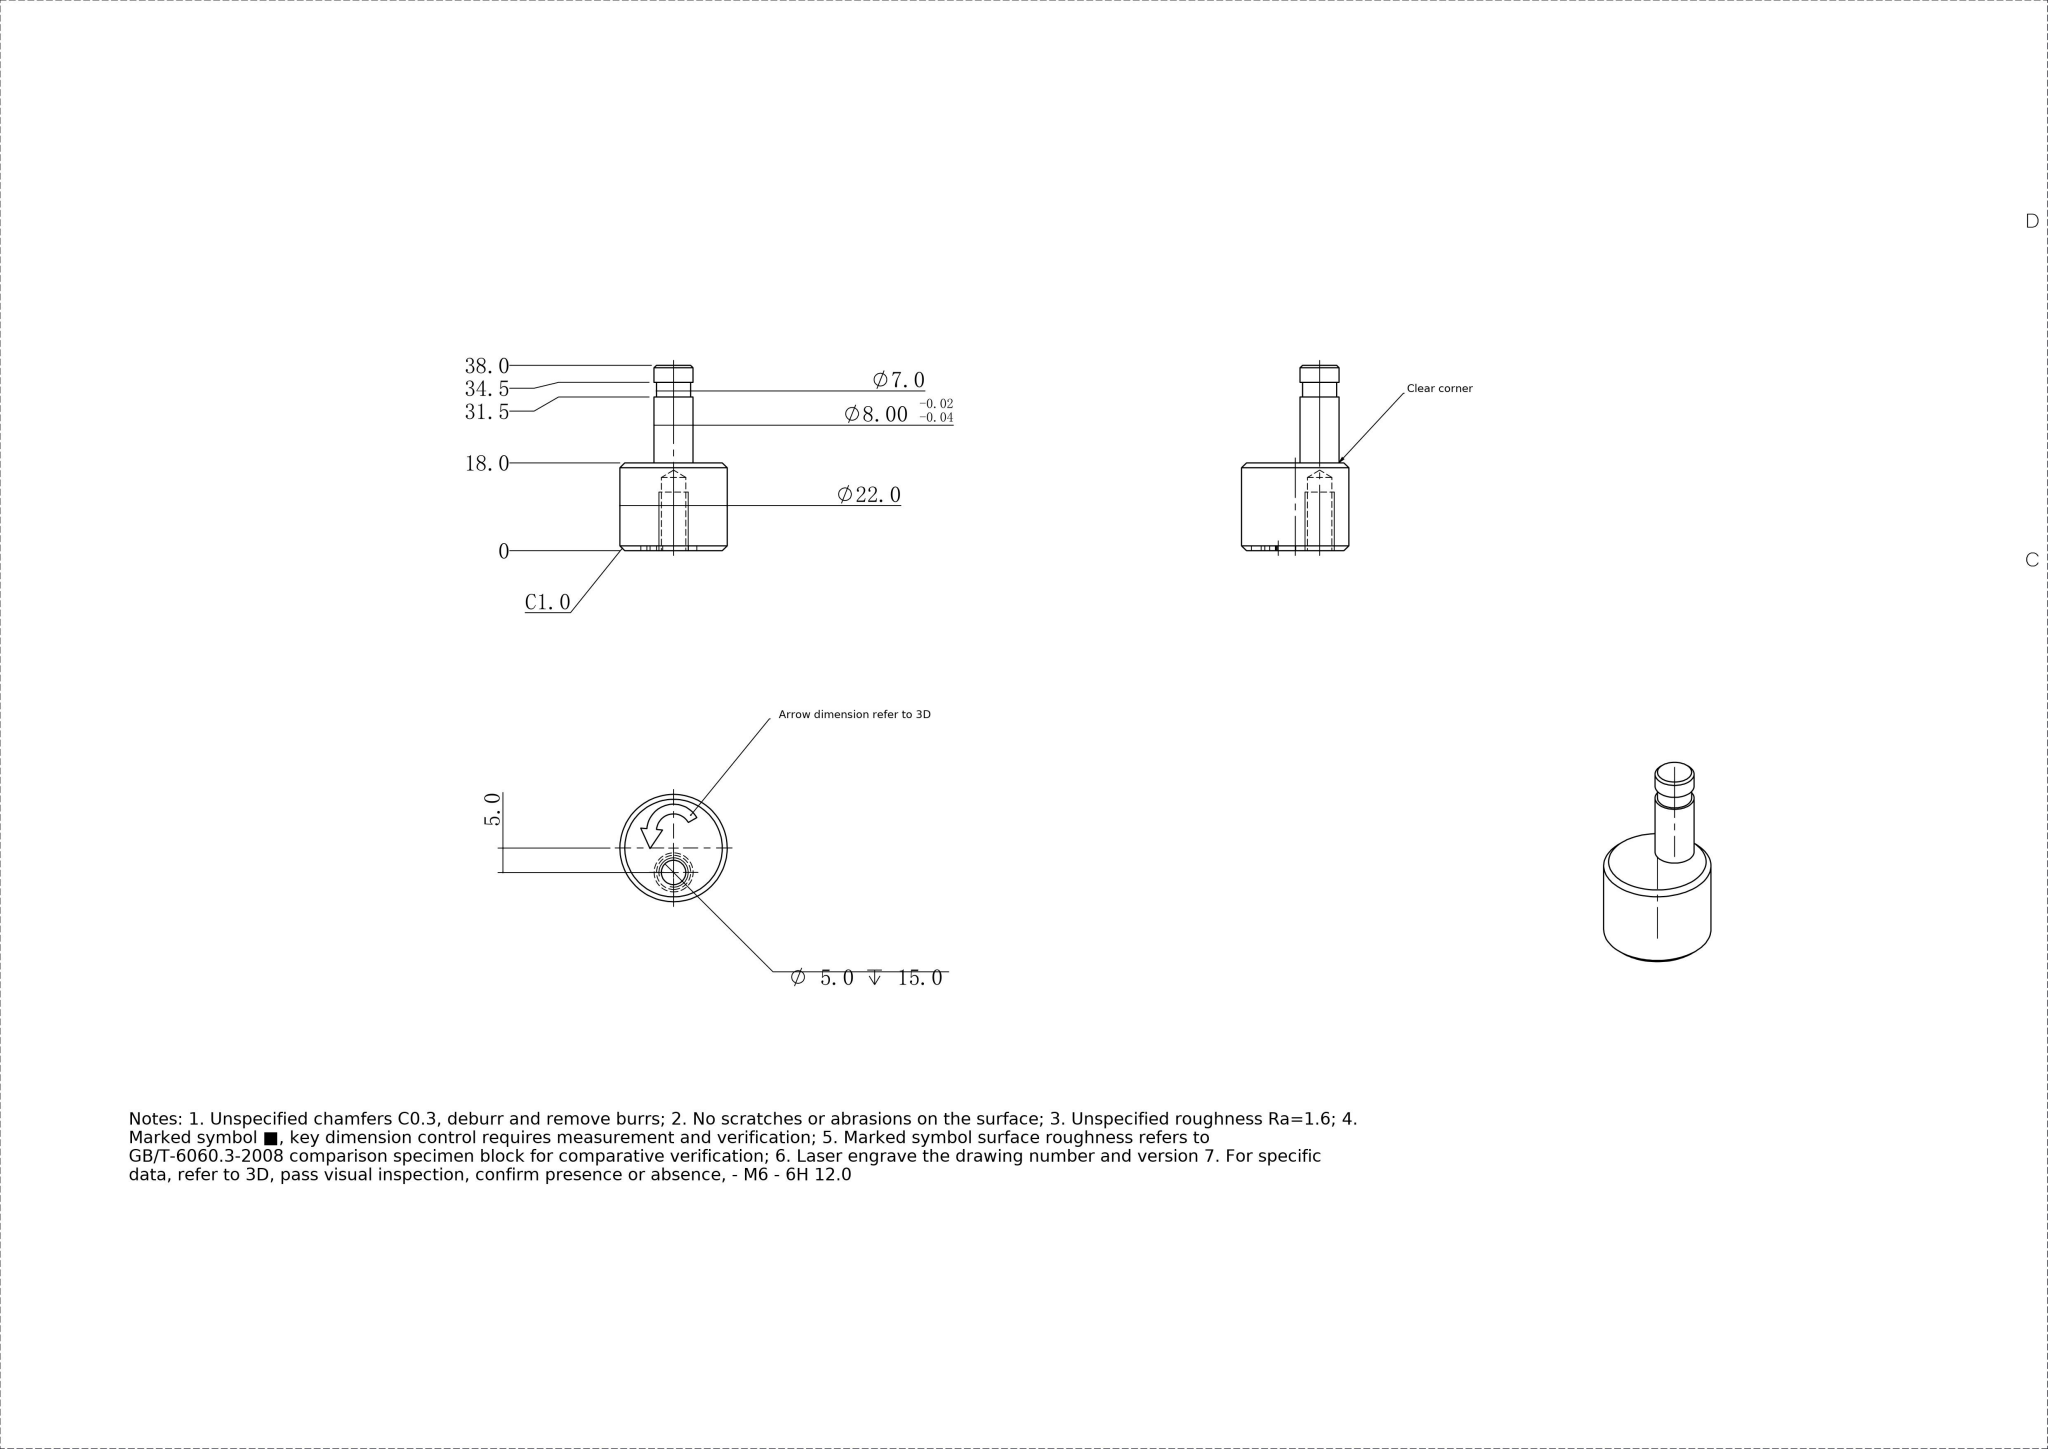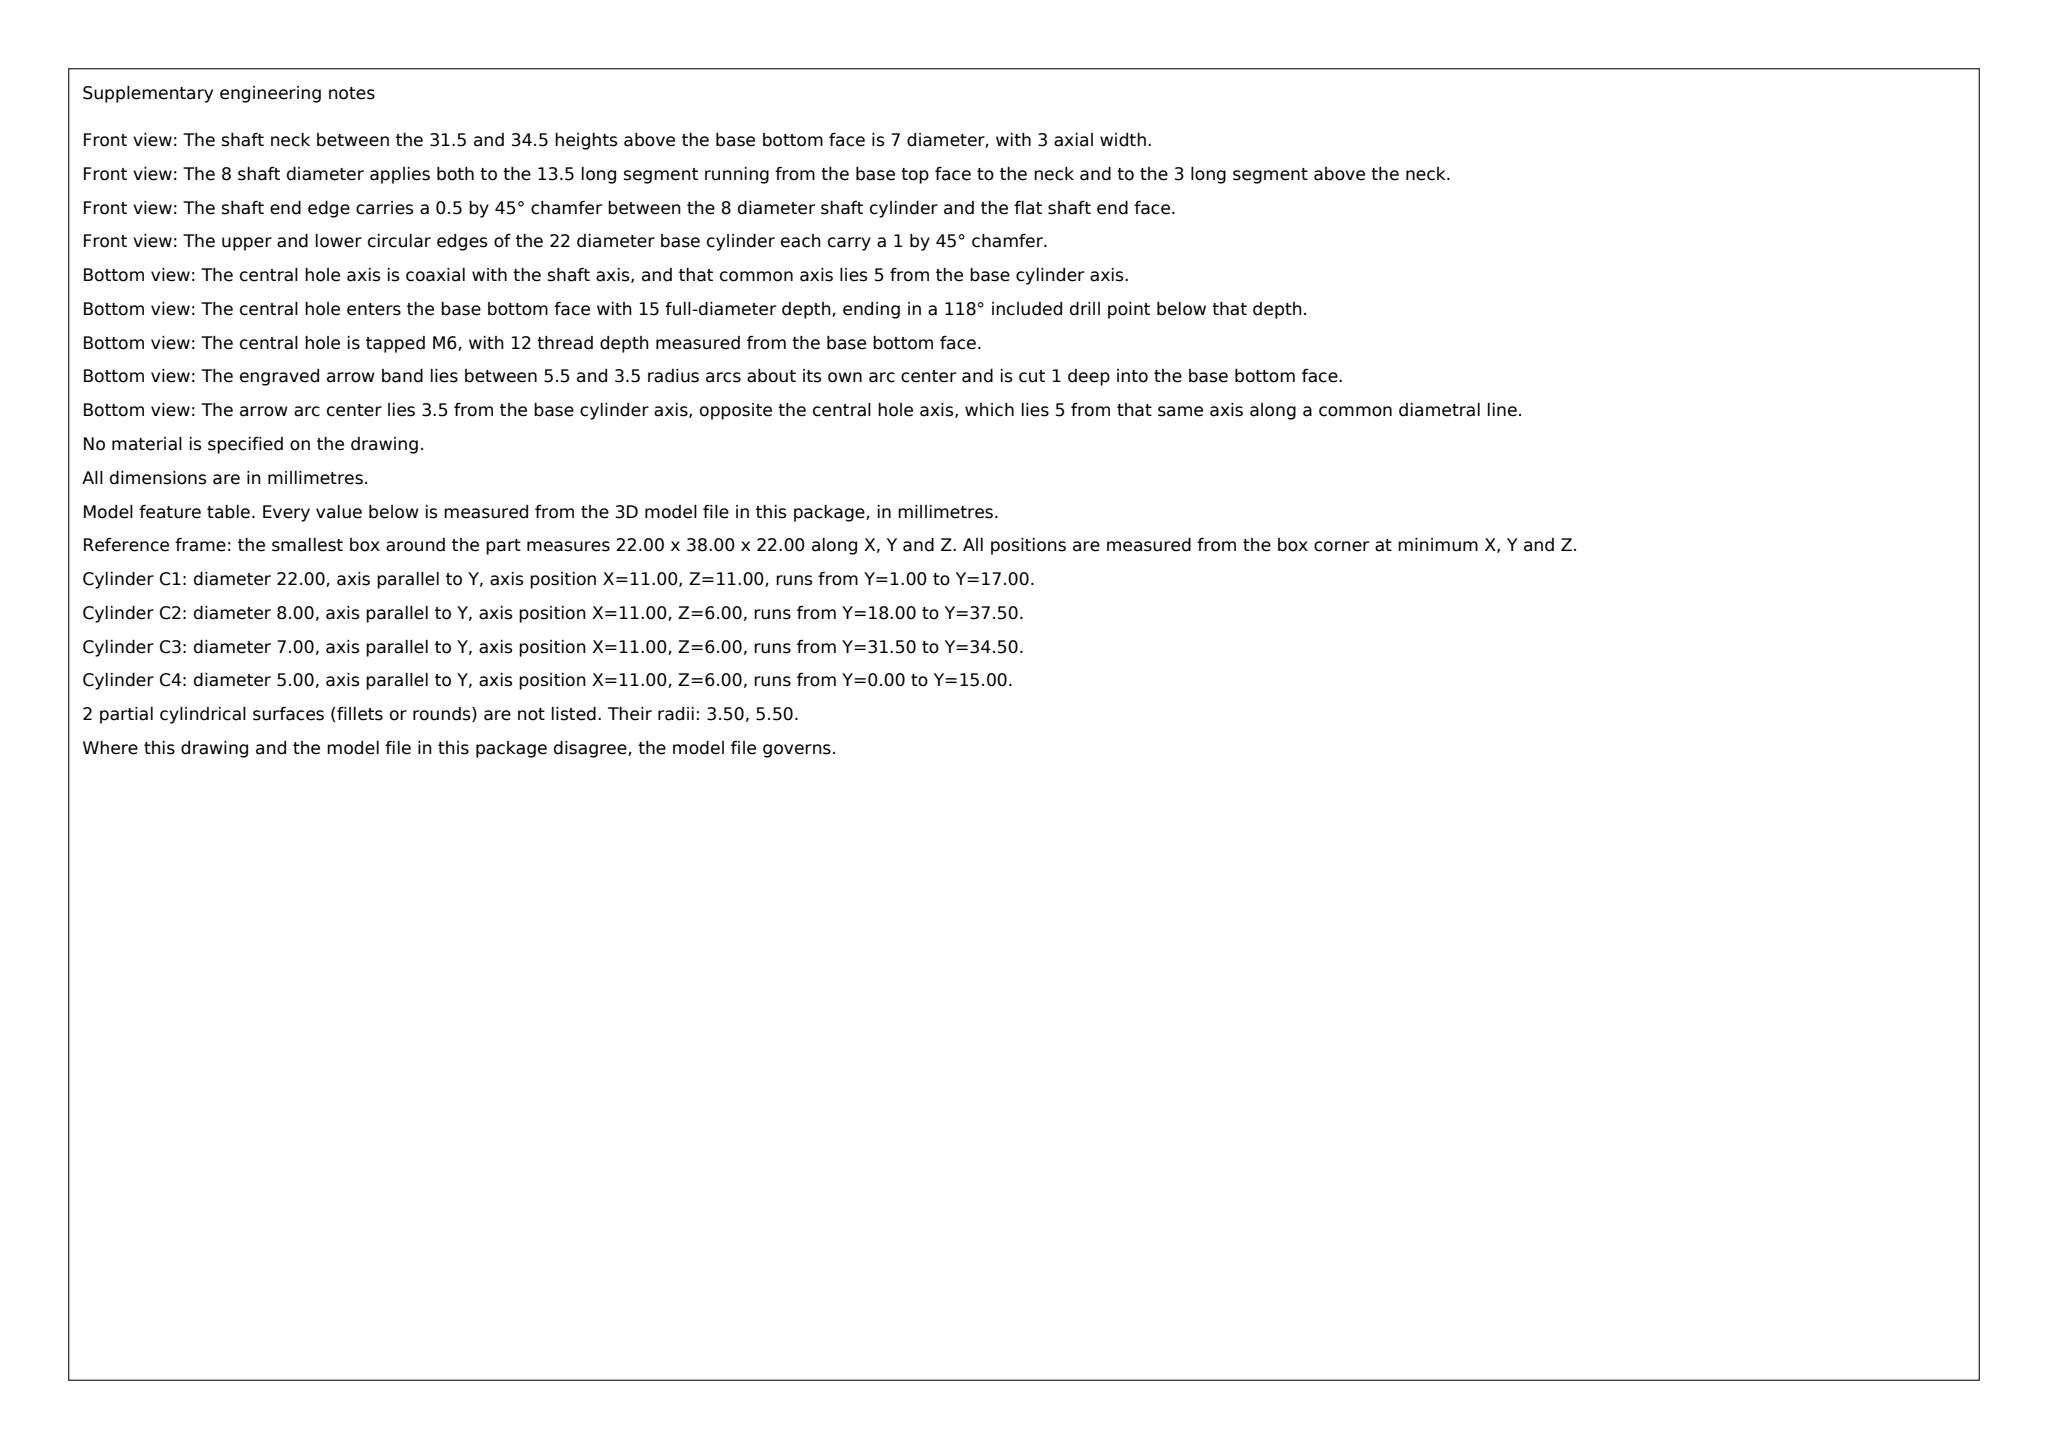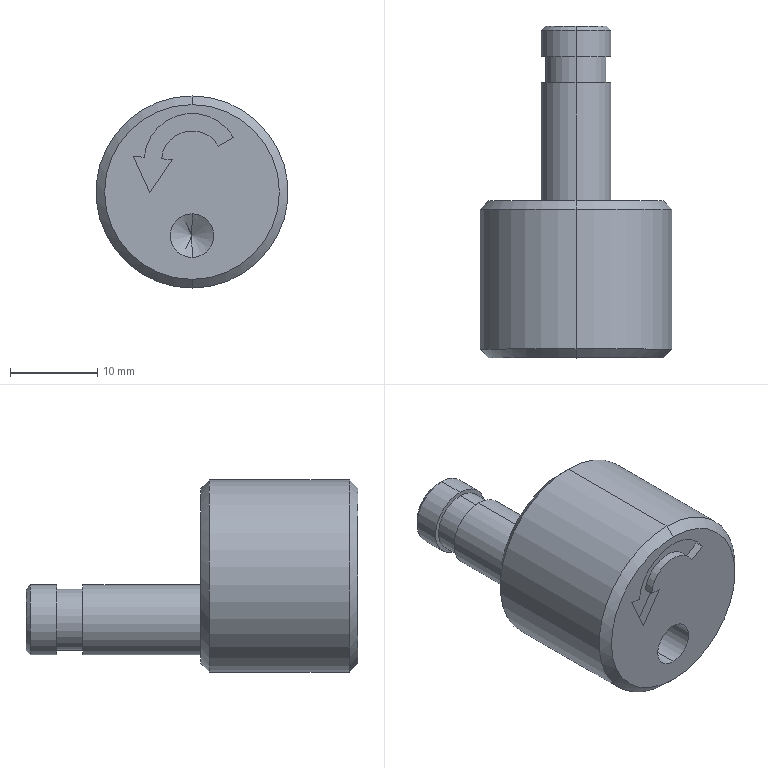Part | SolidWorks | mm | 1 solid | 31 faces | box 22 x 38 x 22 mm | volume 7406 mm3 | cylinder 12 | plane 11 | cone 8 | commonest cylinder face diameters 8 x4 7 x3 5 x2 22 x2 11 x1
Drawing notes:
ARROW ENGRAVING ARC GROOVE: 145° ARC SWEEP, Ø11.0 OUTER / Ø7.0 INNER, DP 1.0 FROM BOTTOM FACE (Y=0 DATUM); ARC CENTRE ON Ø22.0 BODY CENTRELINE, OFFSET 3.5 FROM Ø22.0 AXIS | from the solid: cylinders: concave arc Ø11.0 and convex arc Ø7.0, axis y at (x=11.0, z=14.5), from y=0.0 to 1.0, arc_deg 145
ARROW HEAD: ENGRAVED FLAT-BOTTOM POCKET DP 1.0 FROM BOTTOM FACE (Y=0 DATUM), FLANK FACES AT 24.4° AND 34.4° TO X AXIS, WITHIN 11.5 (X) x 9.1 (Z) ENVELOPE FROM X=4.3, Z=10.9 | from the solid: axis_plane y=1.0 extent x[4.3,15.8] z[10.9,20.0]; inclined_planes angle_to_xyz 24.4/90/65.6 and 34.4/90/55.6, bbox_from [4.3,0,10.9] and [6.2,0,10.9]
2X C1.0 CHAMFER (90° INCLUDED) ON Ø22.0 BODY: BOTTOM EDGE AT Y=0 (Ø20.0 AT FACE) AND TOP EDGE AT Y=18.0 (CHAMFER Y=17.0 TO 18.0), Y=0 BOTTOM FACE DATUM | from the solid: cones: 90° ref_dia 20.0 bbox_from y=0.0 size y 1.0; 90° ref_dia 22.0 bbox_from y=17.0 size y 1.0
build123d program:
from build123d import *

# Parameters (mm, degrees)
SKETCH1_W             = 11
SKETCH1_H             = 18
CUT_EXTRUDE1_DEPTH    = 1
M6_TAPPED_HOLE1_D     = 5
M6_TAPPED_HOLE1_DEPTH = 15
M6_TAPPED_HOLE1_TIP   = 1.502
CHAMFER1_SIZE         = 1
CHAMFER2_SIZE         = 0.5


with BuildPart() as part:
    # Sketch1 → Revolve1 (revolve)
    with BuildSketch(Plane.XY, mode=Mode.PRIVATE) as revolve1_sk:
        with Locations((5.5, 0)):
            Rectangle(SKETCH1_W, SKETCH1_H)
    revolve(revolve1_sk.sketch.rotate(Axis((0, 9, 0), (0, -1, 0)), 270), axis=Axis((0, 9, 0), (0, -1, 0)))

    # Sketch2 → Cut-Extrude1 (cut)
    with BuildSketch(Plane.XZ.offset(9)):
        with BuildLine():
            Line((-6.724, 4.088), (-4.831, -0.09258))
            Line((-4.831, -0.09258), (-2.241, 3.696))
            Line((-2.241, 3.696), (-3.487, 3.805))
            ThreePointArc((-3.487, 3.805), (-0.7575, 6.917), (3.031, 5.25))
            Line((3.031, 5.25), (4.763, 6.25))
            ThreePointArc((4.763, 6.25), (-1.19, 8.87), (-5.479, 3.979))
            Line((-5.479, 3.979), (-6.724, 4.088))
        make_face()
    extrude(amount=-CUT_EXTRUDE1_DEPTH, mode=Mode.SUBTRACT)

    # Sketch3 → Revolve2 (revolve)
    with BuildSketch(Plane.XY.offset(-5), mode=Mode.PRIVATE) as revolve2_sk:
        Polygon((4, 29), (0, 29), (0, 9), (4, 9), (4, 22.5), (3.5, 22.5), (3.5, 25.5), (4, 25.5), align=None)
    revolve(revolve2_sk.sketch.rotate(Axis((0, 29, -5), (0, -1, 0)), 270), axis=Axis((0, 29, -5), (0, -1, 0)))

    # M6 Tapped Hole1
    with Locations(Plane(origin=(0, -9, 0), x_dir=(-1, 0, 0), z_dir=(0, -1, 0))):
        with Locations((0, 5)):
            Hole(M6_TAPPED_HOLE1_D / 2, depth=M6_TAPPED_HOLE1_DEPTH)
            with Locations((0, 0, -(M6_TAPPED_HOLE1_DEPTH + M6_TAPPED_HOLE1_TIP / 2))):  # 118° drill point
                Cone(0, M6_TAPPED_HOLE1_D / 2, M6_TAPPED_HOLE1_TIP, mode=Mode.SUBTRACT)

    # Chamfer1
    chamfer1_edges = [part.edges().sort_by_distance(p)[0] for p in [
        (0, -9, 11),
        (0, 9, 11),
    ]]
    chamfer(chamfer1_edges, length=CHAMFER1_SIZE)

    # Chamfer2
    chamfer2_edges = [part.edges().sort_by_distance(p)[0] for p in [
        (0, 29, -1),
    ]]
    chamfer(chamfer2_edges, length=CHAMFER2_SIZE)


solid = part.part
STEP:
#1=CARTESIAN_POINT('',(0.,29.,-1.5));
#2=VERTEX_POINT('',#1);
#3=CARTESIAN_POINT('',(0.,29.,-8.5));
#4=VERTEX_POINT('',#3);
#5=CARTESIAN_POINT('',(0.,29.,-5.));
#6=DIRECTION('',(0.,1.,0.));
#7=DIRECTION('',(0.,0.,1.));
#8=AXIS2_PLACEMENT_3D('',#5,#6,#7);
#9=CIRCLE('',#8,3.5);
#10=EDGE_CURVE('',#2,#4,#9,.T.);
#11=ORIENTED_EDGE('',*,*,#10,.F.);
#12=CARTESIAN_POINT('',(0.,28.5,-1.));
#13=VERTEX_POINT('',#12);
#14=CARTESIAN_POINT('',(0.,28.5,-1.));
#15=DIRECTION('',(0.,-0.7071,0.7071));
#16=VECTOR('',#15,1000.);
#17=LINE('',#14,#16);
#18=EDGE_CURVE('',#2,#13,#17,.T.);
#19=ORIENTED_EDGE('',*,*,#18,.T.);
#20=CARTESIAN_POINT('',(0.,28.5,-9.));
#21=VERTEX_POINT('',#20);
#22=CARTESIAN_POINT('',(0.,28.5,-5.));
#23=DIRECTION('',(0.,-1.,0.));
#24=DIRECTION('',(0.,0.,1.));
#25=AXIS2_PLACEMENT_3D('',#22,#23,#24);
#26=CIRCLE('',#25,4.);
#27=EDGE_CURVE('',#21,#13,#26,.T.);
#28=ORIENTED_EDGE('',*,*,#27,.F.);
#29=CARTESIAN_POINT('',(0.,28.5,-9.));
#30=DIRECTION('',(0.,-0.7071,-0.7071));
#31=VECTOR('',#30,1000.);
#32=LINE('',#29,#31);
#33=EDGE_CURVE('',#4,#21,#32,.T.);
#34=ORIENTED_EDGE('',*,*,#33,.F.);
#35=EDGE_LOOP('',(#11,#19,#28,#34));
#36=FACE_OUTER_BOUND('',#35,.T.);
#37=CARTESIAN_POINT('',(0.,28.5,-5.));
#38=DIRECTION('',(0.,-1.,0.));
#39=DIRECTION('',(0.,0.,-1.));
#40=AXIS2_PLACEMENT_3D('',#37,#38,#39);
#41=CONICAL_SURFACE('',#40,4.,0.7854);
#42=ADVANCED_FACE('',(#36),#41,.T.);
#43=CARTESIAN_POINT('',(0.,9.,10.));
#44=VERTEX_POINT('',#43);
#45=CARTESIAN_POINT('',(0.,9.,-10.));
#46=VERTEX_POINT('',#45);
#47=CARTESIAN_POINT('',(0.,9.,0.));
#48=DIRECTION('',(0.,1.,0.));
#49=DIRECTION('',(0.,0.,1.));
#50=AXIS2_PLACEMENT_3D('',#47,#48,#49);
#51=CIRCLE('',#50,10.);
#52=EDGE_CURVE('',#44,#46,#51,.T.);
#53=ORIENTED_EDGE('',*,*,#52,.F.);
#54=CARTESIAN_POINT('',(0.,8.,11.));
#55=VERTEX_POINT('',#54);
#56=CARTESIAN_POINT('',(0.,8.,11.));
#57=DIRECTION('',(0.,-0.7071,0.7071));
#58=VECTOR('',#57,1000.);
#59=LINE('',#56,#58);
#60=EDGE_CURVE('',#44,#55,#59,.T.);
#61=ORIENTED_EDGE('',*,*,#60,.T.);
#62=CARTESIAN_POINT('',(0.,8.,-11.));
#63=VERTEX_POINT('',#62);
#64=CARTESIAN_POINT('',(0.,8.,0.));
#65=DIRECTION('',(0.,-1.,0.));
#66=DIRECTION('',(0.,0.,1.));
#67=AXIS2_PLACEMENT_3D('',#64,#65,#66);
#68=CIRCLE('',#67,11.);
#69=EDGE_CURVE('',#63,#55,#68,.T.);
#70=ORIENTED_EDGE('',*,*,#69,.F.);
#71=CARTESIAN_POINT('',(0.,8.,-11.));
#72=DIRECTION('',(0.,-0.7071,-0.7071));
#73=VECTOR('',#72,1000.);
#74=LINE('',#71,#73);
#75=EDGE_CURVE('',#46,#63,#74,.T.);
#76=ORIENTED_EDGE('',*,*,#75,.F.);
#77=EDGE_LOOP('',(#53,#61,#70,#76));
#78=FACE_OUTER_BOUND('',#77,.T.);
#79=CARTESIAN_POINT('',(0.,8.,0.));
#80=DIRECTION('',(0.,-1.,0.));
#81=DIRECTION('',(0.,0.,-1.));
#82=AXIS2_PLACEMENT_3D('',#79,#80,#81);
#83=CONICAL_SURFACE('',#82,11.,0.7854);
#84=ADVANCED_FACE('',(#78),#83,.T.);
#85=CARTESIAN_POINT('',(0.,-9.,-10.));
#86=VERTEX_POINT('',#85);
#87=CARTESIAN_POINT('',(0.,-9.,10.));
#88=VERTEX_POINT('',#87);
#89=CARTESIAN_POINT('',(0.,-9.,0.));
#90=DIRECTION('',(0.,-1.,0.));
#91=DIRECTION('',(0.,0.,-1.));
#92=AXIS2_PLACEMENT_3D('',#89,#90,#91);
#93=CIRCLE('',#92,10.);
#94=EDGE_CURVE('',#86,#88,#93,.T.);
#95=ORIENTED_EDGE('',*,*,#94,.F.);
#96=CARTESIAN_POINT('',(0.,-8.,-11.));
#97=VERTEX_POINT('',#96);
#98=CARTESIAN_POINT('',(0.,-9.,-10.));
#99=DIRECTION('',(0.,0.7071,-0.7071));
#100=VECTOR('',#99,1000.);
#101=LINE('',#98,#100);
#102=EDGE_CURVE('',#86,#97,#101,.T.);
#103=ORIENTED_EDGE('',*,*,#102,.T.);
#104=CARTESIAN_POINT('',(0.,-8.,11.));
#105=VERTEX_POINT('',#104);
#106=CARTESIAN_POINT('',(0.,-8.,0.));
#107=DIRECTION('',(0.,1.,0.));
#108=DIRECTION('',(0.,0.,-1.));
#109=AXIS2_PLACEMENT_3D('',#106,#107,#108);
#110=CIRCLE('',#109,11.);
#111=EDGE_CURVE('',#105,#97,#110,.T.);
#112=ORIENTED_EDGE('',*,*,#111,.F.);
#113=CARTESIAN_POINT('',(0.,-9.,10.));
#114=DIRECTION('',(0.,0.7071,0.7071));
#115=VECTOR('',#114,1000.);
#116=LINE('',#113,#115);
#117=EDGE_CURVE('',#88,#105,#116,.T.);
#118=ORIENTED_EDGE('',*,*,#117,.F.);
#119=EDGE_LOOP('',(#95,#103,#112,#118));
#120=FACE_OUTER_BOUND('',#119,.T.);
#121=CARTESIAN_POINT('',(0.,-9.,0.));
#122=DIRECTION('',(0.,1.,0.));
#123=DIRECTION('',(0.,0.,1.));
#124=AXIS2_PLACEMENT_3D('',#121,#122,#123);
#125=CONICAL_SURFACE('',#124,10.,0.7854);
#126=ADVANCED_FACE('',(#120),#125,.T.);
#127=CARTESIAN_POINT('',(0.,6.,-2.5));
#128=VERTEX_POINT('',#127);
#129=CARTESIAN_POINT('',(0.,6.,-7.5));
#130=VERTEX_POINT('',#129);
#131=CARTESIAN_POINT('',(0.,6.,-5.));
#132=DIRECTION('',(0.,-1.,0.));
#133=DIRECTION('',(0.,0.,-1.));
#134=AXIS2_PLACEMENT_3D('',#131,#132,#133);
#135=CIRCLE('',#134,2.5);
#136=EDGE_CURVE('',#128,#130,#135,.T.);
#137=ORIENTED_EDGE('',*,*,#136,.F.);
#138=CARTESIAN_POINT('',(0.,-9.,-2.5));
#139=VERTEX_POINT('',#138);
#140=CARTESIAN_POINT('',(0.,-9.,-2.5));
#141=DIRECTION('',(0.,-1.,0.));
#142=VECTOR('',#141,1000.);
#143=LINE('',#140,#142);
#144=EDGE_CURVE('',#128,#139,#143,.T.);
#145=ORIENTED_EDGE('',*,*,#144,.T.);
#146=CARTESIAN_POINT('',(0.,-9.,-7.5));
#147=VERTEX_POINT('',#146);
#148=CARTESIAN_POINT('',(0.,-9.,-5.));
#149=DIRECTION('',(0.,-1.,0.));
#150=DIRECTION('',(0.,0.,-1.));
#151=AXIS2_PLACEMENT_3D('',#148,#149,#150);
#152=CIRCLE('',#151,2.5);
#153=EDGE_CURVE('',#139,#147,#152,.T.);
#154=ORIENTED_EDGE('',*,*,#153,.T.);
#155=CARTESIAN_POINT('',(0.,-9.,-7.5));
#156=DIRECTION('',(0.,-1.,0.));
#157=VECTOR('',#156,1000.);
#158=LINE('',#155,#157);
#159=EDGE_CURVE('',#130,#147,#158,.T.);
#160=ORIENTED_EDGE('',*,*,#159,.F.);
#161=EDGE_LOOP('',(#137,#145,#154,#160));
#162=FACE_OUTER_BOUND('',#161,.T.);
#163=CARTESIAN_POINT('',(0.,-9.,-5.));
#164=DIRECTION('',(0.,-1.,0.));
#165=DIRECTION('',(0.,0.,-1.));
#166=AXIS2_PLACEMENT_3D('',#163,#164,#165);
#167=CYLINDRICAL_SURFACE('',#166,2.5);
#168=ADVANCED_FACE('',(#162),#167,.F.);
#169=CARTESIAN_POINT('',(-0.,7.502,-5.));
#170=VERTEX_POINT('',#169);
#171=CARTESIAN_POINT('',(0.,6.,-7.5));
#172=DIRECTION('',(0.,-0.515,-0.8572));
#173=VECTOR('',#172,1000.);
#174=LINE('',#171,#173);
#175=EDGE_CURVE('',#170,#130,#174,.T.);
#176=ORIENTED_EDGE('',*,*,#175,.F.);
#177=CARTESIAN_POINT('',(0.,6.,-2.5));
#178=DIRECTION('',(0.,-0.515,0.8572));
#179=VECTOR('',#178,1000.);
#180=LINE('',#177,#179);
#181=EDGE_CURVE('',#170,#128,#180,.T.);
#182=ORIENTED_EDGE('',*,*,#181,.T.);
#183=ORIENTED_EDGE('',*,*,#136,.T.);
#184=EDGE_LOOP('',(#176,#182,#183));
#185=FACE_OUTER_BOUND('',#184,.T.);
#186=CARTESIAN_POINT('',(0.,6.,-5.));
#187=DIRECTION('',(0.,-1.,0.));
#188=DIRECTION('',(0.,0.,-1.));
#189=AXIS2_PLACEMENT_3D('',#186,#187,#188);
#190=CONICAL_SURFACE('',#189,2.5,1.03);
#191=ADVANCED_FACE('',(#185),#190,.F.);
#192=CARTESIAN_POINT('',(0.,25.5,-8.5));
#193=VERTEX_POINT('',#192);
#194=CARTESIAN_POINT('',(0.,25.5,-1.5));
#195=VERTEX_POINT('',#194);
#196=CARTESIAN_POINT('',(0.,25.5,-5.));
#197=DIRECTION('',(0.,-1.,0.));
#198=DIRECTION('',(0.,0.,-1.));
#199=AXIS2_PLACEMENT_3D('',#196,#197,#198);
#200=CIRCLE('',#199,3.5);
#201=EDGE_CURVE('',#193,#195,#200,.T.);
#202=ORIENTED_EDGE('',*,*,#201,.T.);
#203=CARTESIAN_POINT('',(0.,22.5,-1.5));
#204=VERTEX_POINT('',#203);
#205=CARTESIAN_POINT('',(0.,29.,-1.5));
#206=DIRECTION('',(0.,-1.,0.));
#207=VECTOR('',#206,1000.);
#208=LINE('',#205,#207);
#209=EDGE_CURVE('',#195,#204,#208,.T.);
#210=ORIENTED_EDGE('',*,*,#209,.T.);
#211=CARTESIAN_POINT('',(0.,22.5,-8.5));
#212=VERTEX_POINT('',#211);
#213=CARTESIAN_POINT('',(0.,22.5,-5.));
#214=DIRECTION('',(0.,-1.,0.));
#215=DIRECTION('',(0.,0.,-1.));
#216=AXIS2_PLACEMENT_3D('',#213,#214,#215);
#217=CIRCLE('',#216,3.5);
#218=EDGE_CURVE('',#212,#204,#217,.T.);
#219=ORIENTED_EDGE('',*,*,#218,.F.);
#220=CARTESIAN_POINT('',(0.,29.,-8.5));
#221=DIRECTION('',(0.,-1.,0.));
#222=VECTOR('',#221,1000.);
#223=LINE('',#220,#222);
#224=EDGE_CURVE('',#193,#212,#223,.T.);
#225=ORIENTED_EDGE('',*,*,#224,.F.);
#226=EDGE_LOOP('',(#202,#210,#219,#225));
#227=FACE_OUTER_BOUND('',#226,.T.);
#228=CARTESIAN_POINT('',(0.,29.,-5.));
#229=DIRECTION('',(0.,-1.,0.));
#230=DIRECTION('',(0.,0.,-1.));
#231=AXIS2_PLACEMENT_3D('',#228,#229,#230);
#232=CYLINDRICAL_SURFACE('',#231,3.5);
#233=ADVANCED_FACE('',(#227),#232,.T.);
#234=CARTESIAN_POINT('',(0.,22.5,-9.));
#235=VERTEX_POINT('',#234);
#236=CARTESIAN_POINT('',(0.,22.5,-1.));
#237=VERTEX_POINT('',#236);
#238=CARTESIAN_POINT('',(0.,22.5,-5.));
#239=DIRECTION('',(0.,-1.,0.));
#240=DIRECTION('',(0.,0.,-1.));
#241=AXIS2_PLACEMENT_3D('',#238,#239,#240);
#242=CIRCLE('',#241,4.);
#243=EDGE_CURVE('',#235,#237,#242,.T.);
#244=ORIENTED_EDGE('',*,*,#243,.T.);
#245=CARTESIAN_POINT('',(0.,9.,-1.));
#246=VERTEX_POINT('',#245);
#247=CARTESIAN_POINT('',(0.,29.,-1.));
#248=DIRECTION('',(0.,-1.,0.));
#249=VECTOR('',#248,1000.);
#250=LINE('',#247,#249);
#251=EDGE_CURVE('',#237,#246,#250,.T.);
#252=ORIENTED_EDGE('',*,*,#251,.T.);
#253=CARTESIAN_POINT('',(0.,9.,-9.));
#254=VERTEX_POINT('',#253);
#255=CARTESIAN_POINT('',(0.,9.,-5.));
#256=DIRECTION('',(0.,-1.,0.));
#257=DIRECTION('',(0.,0.,-1.));
#258=AXIS2_PLACEMENT_3D('',#255,#256,#257);
#259=CIRCLE('',#258,4.);
#260=EDGE_CURVE('',#254,#246,#259,.T.);
#261=ORIENTED_EDGE('',*,*,#260,.F.);
#262=CARTESIAN_POINT('',(0.,29.,-9.));
#263=DIRECTION('',(0.,-1.,0.));
#264=VECTOR('',#263,1000.);
#265=LINE('',#262,#264);
#266=EDGE_CURVE('',#235,#254,#265,.T.);
#267=ORIENTED_EDGE('',*,*,#266,.F.);
#268=EDGE_LOOP('',(#244,#252,#261,#267));
#269=FACE_OUTER_BOUND('',#268,.T.);
#270=CARTESIAN_POINT('',(0.,29.,-5.));
#271=DIRECTION('',(0.,-1.,0.));
#272=DIRECTION('',(0.,0.,-1.));
#273=AXIS2_PLACEMENT_3D('',#270,#271,#272);
#274=CYLINDRICAL_SURFACE('',#273,4.);
#275=ADVANCED_FACE('',(#269),#274,.T.);
#276=ORIENTED_EDGE('',*,*,#27,.T.);
#277=CARTESIAN_POINT('',(0.,25.5,-1.));
#278=VERTEX_POINT('',#277);
#279=CARTESIAN_POINT('',(0.,29.,-1.));
#280=DIRECTION('',(0.,-1.,0.));
#281=VECTOR('',#280,1000.);
#282=LINE('',#279,#281);
#283=EDGE_CURVE('',#13,#278,#282,.T.);
#284=ORIENTED_EDGE('',*,*,#283,.T.);
#285=CARTESIAN_POINT('',(0.,25.5,-9.));
#286=VERTEX_POINT('',#285);
#287=CARTESIAN_POINT('',(0.,25.5,-5.));
#288=DIRECTION('',(0.,-1.,0.));
#289=DIRECTION('',(0.,0.,-1.));
#290=AXIS2_PLACEMENT_3D('',#287,#288,#289);
#291=CIRCLE('',#290,4.);
#292=EDGE_CURVE('',#286,#278,#291,.T.);
#293=ORIENTED_EDGE('',*,*,#292,.F.);
#294=CARTESIAN_POINT('',(0.,29.,-9.));
#295=DIRECTION('',(0.,-1.,0.));
#296=VECTOR('',#295,1000.);
#297=LINE('',#294,#296);
#298=EDGE_CURVE('',#21,#286,#297,.T.);
#299=ORIENTED_EDGE('',*,*,#298,.F.);
#300=EDGE_LOOP('',(#276,#284,#293,#299));
#301=FACE_OUTER_BOUND('',#300,.T.);
#302=CARTESIAN_POINT('',(0.,29.,-5.));
#303=DIRECTION('',(0.,-1.,0.));
#304=DIRECTION('',(0.,0.,-1.));
#305=AXIS2_PLACEMENT_3D('',#302,#303,#304);
#306=CYLINDRICAL_SURFACE('',#305,4.);
#307=ADVANCED_FACE('',(#301),#306,.T.);
#308=ORIENTED_EDGE('',*,*,#69,.T.);
#309=CARTESIAN_POINT('',(0.,9.,11.));
#310=DIRECTION('',(0.,-1.,0.));
#311=VECTOR('',#310,1000.);
#312=LINE('',#309,#311);
#313=EDGE_CURVE('',#55,#105,#312,.T.);
#314=ORIENTED_EDGE('',*,*,#313,.T.);
#315=ORIENTED_EDGE('',*,*,#111,.T.);
#316=CARTESIAN_POINT('',(0.,9.,-11.));
#317=DIRECTION('',(0.,-1.,0.));
#318=VECTOR('',#317,1000.);
#319=LINE('',#316,#318);
#320=EDGE_CURVE('',#63,#97,#319,.T.);
#321=ORIENTED_EDGE('',*,*,#320,.F.);
#322=EDGE_LOOP('',(#308,#314,#315,#321));
#323=FACE_OUTER_BOUND('',#322,.T.);
#324=CARTESIAN_POINT('',(0.,9.,0.));
#325=DIRECTION('',(0.,-1.,0.));
#326=DIRECTION('',(0.,0.,-1.));
#327=AXIS2_PLACEMENT_3D('',#324,#325,#326);
#328=CYLINDRICAL_SURFACE('',#327,11.);
#329=ADVANCED_FACE('',(#323),#328,.T.);
#330=ORIENTED_EDGE('',*,*,#313,.F.);
#331=CARTESIAN_POINT('',(0.,8.,0.));
#332=DIRECTION('',(0.,-1.,0.));
#333=DIRECTION('',(0.,0.,1.));
#334=AXIS2_PLACEMENT_3D('',#331,#332,#333);
#335=CIRCLE('',#334,11.);
#336=EDGE_CURVE('',#55,#63,#335,.T.);
#337=ORIENTED_EDGE('',*,*,#336,.T.);
#338=ORIENTED_EDGE('',*,*,#320,.T.);
#339=CARTESIAN_POINT('',(0.,-8.,0.));
#340=DIRECTION('',(0.,1.,0.));
#341=DIRECTION('',(0.,0.,-1.));
#342=AXIS2_PLACEMENT_3D('',#339,#340,#341);
#343=CIRCLE('',#342,11.);
#344=EDGE_CURVE('',#97,#105,#343,.T.);
#345=ORIENTED_EDGE('',*,*,#344,.T.);
#346=EDGE_LOOP('',(#330,#337,#338,#345));
#347=FACE_OUTER_BOUND('',#346,.T.);
#348=CARTESIAN_POINT('',(0.,9.,0.));
#349=DIRECTION('',(0.,-1.,0.));
#350=DIRECTION('',(0.,0.,-1.));
#351=AXIS2_PLACEMENT_3D('',#348,#349,#350);
#352=CYLINDRICAL_SURFACE('',#351,11.);
#353=ADVANCED_FACE('',(#347),#352,.T.);
#354=CARTESIAN_POINT('',(0.,9.,0.));
#355=DIRECTION('',(0.,1.,0.));
#356=DIRECTION('',(0.,0.,1.));
#357=AXIS2_PLACEMENT_3D('',#354,#355,#356);
#358=CIRCLE('',#357,10.);
#359=EDGE_CURVE('',#46,#44,#358,.T.);
#360=ORIENTED_EDGE('',*,*,#359,.T.);
#361=ORIENTED_EDGE('',*,*,#52,.T.);
#362=EDGE_LOOP('',(#360,#361));
#363=FACE_OUTER_BOUND('',#362,.T.);
#364=ORIENTED_EDGE('',*,*,#260,.T.);
#365=CARTESIAN_POINT('',(0.,9.,-5.));
#366=DIRECTION('',(0.,-1.,0.));
#367=DIRECTION('',(0.,0.,-1.));
#368=AXIS2_PLACEMENT_3D('',#365,#366,#367);
#369=CIRCLE('',#368,4.);
#370=EDGE_CURVE('',#246,#254,#369,.T.);
#371=ORIENTED_EDGE('',*,*,#370,.T.);
#372=EDGE_LOOP('',(#364,#371));
#373=FACE_BOUND('',#372,.T.);
#374=CARTESIAN_POINT('',(11.,9.,0.));
#375=DIRECTION('',(0.,1.,0.));
#376=DIRECTION('',(0.,0.,1.));
#377=AXIS2_PLACEMENT_3D('',#374,#375,#376);
#378=PLANE('',#377);
#379=ADVANCED_FACE('',(#363,#373),#378,.T.);
#380=CARTESIAN_POINT('',(0.,-9.,0.));
#381=DIRECTION('',(0.,-1.,0.));
#382=DIRECTION('',(0.,0.,-1.));
#383=AXIS2_PLACEMENT_3D('',#380,#381,#382);
#384=CIRCLE('',#383,10.);
#385=EDGE_CURVE('',#88,#86,#384,.T.);
#386=ORIENTED_EDGE('',*,*,#385,.T.);
#387=ORIENTED_EDGE('',*,*,#94,.T.);
#388=EDGE_LOOP('',(#386,#387));
#389=FACE_OUTER_BOUND('',#388,.T.);
#390=CARTESIAN_POINT('',(0.,-9.,-5.));
#391=DIRECTION('',(0.,-1.,0.));
#392=DIRECTION('',(0.,0.,-1.));
#393=AXIS2_PLACEMENT_3D('',#390,#391,#392);
#394=CIRCLE('',#393,2.5);
#395=EDGE_CURVE('',#147,#139,#394,.T.);
#396=ORIENTED_EDGE('',*,*,#395,.F.);
#397=ORIENTED_EDGE('',*,*,#153,.F.);
#398=EDGE_LOOP('',(#396,#397));
#399=FACE_BOUND('',#398,.T.);
#400=CARTESIAN_POINT('',(-5.479,-9.,3.979));
#401=VERTEX_POINT('',#400);
#402=CARTESIAN_POINT('',(-6.724,-9.,4.088));
#403=VERTEX_POINT('',#402);
#404=CARTESIAN_POINT('',(-5.479,-9.,3.979));
#405=DIRECTION('',(-0.9962,0.,0.08716));
#406=VECTOR('',#405,1000.);
#407=LINE('',#404,#406);
#408=EDGE_CURVE('',#401,#403,#407,.T.);
#409=ORIENTED_EDGE('',*,*,#408,.F.);
#410=CARTESIAN_POINT('',(4.763,-9.,6.25));
#411=VERTEX_POINT('',#410);
#412=CARTESIAN_POINT('',(-0.,-9.,3.5));
#413=DIRECTION('',(0.,-1.,0.));
#414=DIRECTION('',(0.,0.,-1.));
#415=AXIS2_PLACEMENT_3D('',#412,#413,#414);
#416=CIRCLE('',#415,5.5);
#417=EDGE_CURVE('',#411,#401,#416,.T.);
#418=ORIENTED_EDGE('',*,*,#417,.F.);
#419=CARTESIAN_POINT('',(3.031,-9.,5.25));
#420=VERTEX_POINT('',#419);
#421=CARTESIAN_POINT('',(3.031,-9.,5.25));
#422=DIRECTION('',(0.866,0.,0.5));
#423=VECTOR('',#422,1000.);
#424=LINE('',#421,#423);
#425=EDGE_CURVE('',#420,#411,#424,.T.);
#426=ORIENTED_EDGE('',*,*,#425,.F.);
#427=CARTESIAN_POINT('',(-3.487,-9.,3.805));
#428=VERTEX_POINT('',#427);
#429=CARTESIAN_POINT('',(-0.,-9.,3.5));
#430=DIRECTION('',(0.,1.,0.));
#431=DIRECTION('',(0.,0.,1.));
#432=AXIS2_PLACEMENT_3D('',#429,#430,#431);
#433=CIRCLE('',#432,3.5);
#434=EDGE_CURVE('',#428,#420,#433,.T.);
#435=ORIENTED_EDGE('',*,*,#434,.F.);
#436=CARTESIAN_POINT('',(-2.241,-9.,3.696));
#437=VERTEX_POINT('',#436);
#438=CARTESIAN_POINT('',(-2.241,-9.,3.696));
#439=DIRECTION('',(-0.9962,0.,0.08716));
#440=VECTOR('',#439,1000.);
#441=LINE('',#438,#440);
#442=EDGE_CURVE('',#437,#428,#441,.T.);
#443=ORIENTED_EDGE('',*,*,#442,.F.);
#444=CARTESIAN_POINT('',(-4.831,-9.,-0.09258));
#445=VERTEX_POINT('',#444);
#446=CARTESIAN_POINT('',(-4.831,-9.,-0.09258));
#447=DIRECTION('',(0.5644,0.,0.8255));
#448=VECTOR('',#447,1000.);
#449=LINE('',#446,#448);
#450=EDGE_CURVE('',#445,#437,#449,.T.);
#451=ORIENTED_EDGE('',*,*,#450,.F.);
#452=CARTESIAN_POINT('',(-6.724,-9.,4.088));
#453=DIRECTION('',(0.4124,0.,-0.911));
#454=VECTOR('',#453,1000.);
#455=LINE('',#452,#454);
#456=EDGE_CURVE('',#403,#445,#455,.T.);
#457=ORIENTED_EDGE('',*,*,#456,.F.);
#458=EDGE_LOOP('',(#409,#418,#426,#435,#443,#451,#457));
#459=FACE_BOUND('',#458,.T.);
#460=CARTESIAN_POINT('',(0.,-9.,0.));
#461=DIRECTION('',(0.,-1.,0.));
#462=DIRECTION('',(0.,0.,-1.));
#463=AXIS2_PLACEMENT_3D('',#460,#461,#462);
#464=PLANE('',#463);
#465=ADVANCED_FACE('',(#389,#399,#459),#464,.T.);
#466=ORIENTED_EDGE('',*,*,#408,.T.);
#467=CARTESIAN_POINT('',(-6.724,-8.,4.088));
#468=VERTEX_POINT('',#467);
#469=CARTESIAN_POINT('',(-6.724,-8.,4.088));
#470=DIRECTION('',(0.,-1.,0.));
#471=VECTOR('',#470,1000.);
#472=LINE('',#469,#471);
#473=EDGE_CURVE('',#468,#403,#472,.T.);
#474=ORIENTED_EDGE('',*,*,#473,.F.);
#475=CARTESIAN_POINT('',(-5.479,-8.,3.979));
#476=VERTEX_POINT('',#475);
#477=CARTESIAN_POINT('',(-5.479,-8.,3.979));
#478=DIRECTION('',(-0.9962,0.,0.08716));
#479=VECTOR('',#478,1000.);
#480=LINE('',#477,#479);
#481=EDGE_CURVE('',#476,#468,#480,.T.);
#482=ORIENTED_EDGE('',*,*,#481,.F.);
#483=CARTESIAN_POINT('',(-5.479,-8.,3.979));
#484=DIRECTION('',(0.,-1.,0.));
#485=VECTOR('',#484,1000.);
#486=LINE('',#483,#485);
#487=EDGE_CURVE('',#476,#401,#486,.T.);
#488=ORIENTED_EDGE('',*,*,#487,.T.);
#489=EDGE_LOOP('',(#466,#474,#482,#488));
#490=FACE_OUTER_BOUND('',#489,.T.);
#491=CARTESIAN_POINT('',(-5.479,-8.,3.979));
#492=DIRECTION('',(0.08716,0.,0.9962));
#493=DIRECTION('',(0.9962,0.,-0.08716));
#494=AXIS2_PLACEMENT_3D('',#491,#492,#493);
#495=PLANE('',#494);
#496=ADVANCED_FACE('',(#490),#495,.F.);
#497=ORIENTED_EDGE('',*,*,#417,.T.);
#498=ORIENTED_EDGE('',*,*,#487,.F.);
#499=CARTESIAN_POINT('',(4.763,-8.,6.25));
#500=VERTEX_POINT('',#499);
#501=CARTESIAN_POINT('',(-0.,-8.,3.5));
#502=DIRECTION('',(0.,-1.,0.));
#503=DIRECTION('',(0.,0.,-1.));
#504=AXIS2_PLACEMENT_3D('',#501,#502,#503);
#505=CIRCLE('',#504,5.5);
#506=EDGE_CURVE('',#500,#476,#505,.T.);
#507=ORIENTED_EDGE('',*,*,#506,.F.);
#508=CARTESIAN_POINT('',(4.763,-8.,6.25));
#509=DIRECTION('',(0.,-1.,0.));
#510=VECTOR('',#509,1000.);
#511=LINE('',#508,#510);
#512=EDGE_CURVE('',#500,#411,#511,.T.);
#513=ORIENTED_EDGE('',*,*,#512,.T.);
#514=EDGE_LOOP('',(#497,#498,#507,#513));
#515=FACE_OUTER_BOUND('',#514,.T.);
#516=CARTESIAN_POINT('',(-0.,-8.,3.5));
#517=DIRECTION('',(0.,-1.,0.));
#518=DIRECTION('',(0.,0.,-1.));
#519=AXIS2_PLACEMENT_3D('',#516,#517,#518);
#520=CYLINDRICAL_SURFACE('',#519,5.5);
#521=ADVANCED_FACE('',(#515),#520,.F.);
#522=ORIENTED_EDGE('',*,*,#425,.T.);
#523=ORIENTED_EDGE('',*,*,#512,.F.);
#524=CARTESIAN_POINT('',(3.031,-8.,5.25));
#525=VERTEX_POINT('',#524);
#526=CARTESIAN_POINT('',(3.031,-8.,5.25));
#527=DIRECTION('',(0.866,0.,0.5));
#528=VECTOR('',#527,1000.);
#529=LINE('',#526,#528);
#530=EDGE_CURVE('',#525,#500,#529,.T.);
#531=ORIENTED_EDGE('',*,*,#530,.F.);
#532=CARTESIAN_POINT('',(3.031,-8.,5.25));
#533=DIRECTION('',(0.,-1.,0.));
#534=VECTOR('',#533,1000.);
#535=LINE('',#532,#534);
#536=EDGE_CURVE('',#525,#420,#535,.T.);
#537=ORIENTED_EDGE('',*,*,#536,.T.);
#538=EDGE_LOOP('',(#522,#523,#531,#537));
#539=FACE_OUTER_BOUND('',#538,.T.);
#540=CARTESIAN_POINT('',(3.031,-8.,5.25));
#541=DIRECTION('',(0.5,0.,-0.866));
#542=DIRECTION('',(-0.866,0.,-0.5));
#543=AXIS2_PLACEMENT_3D('',#540,#541,#542);
#544=PLANE('',#543);
#545=ADVANCED_FACE('',(#539),#544,.F.);
#546=ORIENTED_EDGE('',*,*,#434,.T.);
#547=ORIENTED_EDGE('',*,*,#536,.F.);
#548=CARTESIAN_POINT('',(-3.487,-8.,3.805));
#549=VERTEX_POINT('',#548);
#550=CARTESIAN_POINT('',(-0.,-8.,3.5));
#551=DIRECTION('',(0.,1.,0.));
#552=DIRECTION('',(0.,0.,1.));
#553=AXIS2_PLACEMENT_3D('',#550,#551,#552);
#554=CIRCLE('',#553,3.5);
#555=EDGE_CURVE('',#549,#525,#554,.T.);
#556=ORIENTED_EDGE('',*,*,#555,.F.);
#557=CARTESIAN_POINT('',(-3.487,-8.,3.805));
#558=DIRECTION('',(0.,-1.,0.));
#559=VECTOR('',#558,1000.);
#560=LINE('',#557,#559);
#561=EDGE_CURVE('',#549,#428,#560,.T.);
#562=ORIENTED_EDGE('',*,*,#561,.T.);
#563=EDGE_LOOP('',(#546,#547,#556,#562));
#564=FACE_OUTER_BOUND('',#563,.T.);
#565=CARTESIAN_POINT('',(-0.,-8.,3.5));
#566=DIRECTION('',(0.,-1.,0.));
#567=DIRECTION('',(0.,0.,-1.));
#568=AXIS2_PLACEMENT_3D('',#565,#566,#567);
#569=CYLINDRICAL_SURFACE('',#568,3.5);
#570=ADVANCED_FACE('',(#564),#569,.T.);
#571=ORIENTED_EDGE('',*,*,#442,.T.);
#572=ORIENTED_EDGE('',*,*,#561,.F.);
#573=CARTESIAN_POINT('',(-2.241,-8.,3.696));
#574=VERTEX_POINT('',#573);
#575=CARTESIAN_POINT('',(-2.241,-8.,3.696));
#576=DIRECTION('',(-0.9962,0.,0.08716));
#577=VECTOR('',#576,1000.);
#578=LINE('',#575,#577);
#579=EDGE_CURVE('',#574,#549,#578,.T.);
#580=ORIENTED_EDGE('',*,*,#579,.F.);
#581=CARTESIAN_POINT('',(-2.241,-8.,3.696));
#582=DIRECTION('',(0.,-1.,0.));
#583=VECTOR('',#582,1000.);
#584=LINE('',#581,#583);
#585=EDGE_CURVE('',#574,#437,#584,.T.);
#586=ORIENTED_EDGE('',*,*,#585,.T.);
#587=EDGE_LOOP('',(#571,#572,#580,#586));
#588=FACE_OUTER_BOUND('',#587,.T.);
#589=CARTESIAN_POINT('',(-2.241,-8.,3.696));
#590=DIRECTION('',(0.08716,0.,0.9962));
#591=DIRECTION('',(0.9962,0.,-0.08716));
#592=AXIS2_PLACEMENT_3D('',#589,#590,#591);
#593=PLANE('',#592);
#594=ADVANCED_FACE('',(#588),#593,.F.);
#595=ORIENTED_EDGE('',*,*,#450,.T.);
#596=ORIENTED_EDGE('',*,*,#585,.F.);
#597=CARTESIAN_POINT('',(-4.831,-8.,-0.09258));
#598=VERTEX_POINT('',#597);
#599=CARTESIAN_POINT('',(-4.831,-8.,-0.09258));
#600=DIRECTION('',(0.5644,0.,0.8255));
#601=VECTOR('',#600,1000.);
#602=LINE('',#599,#601);
#603=EDGE_CURVE('',#598,#574,#602,.T.);
#604=ORIENTED_EDGE('',*,*,#603,.F.);
#605=CARTESIAN_POINT('',(-4.831,-8.,-0.09258));
#606=DIRECTION('',(0.,-1.,0.));
#607=VECTOR('',#606,1000.);
#608=LINE('',#605,#607);
#609=EDGE_CURVE('',#598,#445,#608,.T.);
#610=ORIENTED_EDGE('',*,*,#609,.T.);
#611=EDGE_LOOP('',(#595,#596,#604,#610));
#612=FACE_OUTER_BOUND('',#611,.T.);
#613=CARTESIAN_POINT('',(-4.831,-8.,-0.09258));
#614=DIRECTION('',(0.8255,0.,-0.5644));
#615=DIRECTION('',(-0.5644,0.,-0.8255));
#616=AXIS2_PLACEMENT_3D('',#613,#614,#615);
#617=PLANE('',#616);
#618=ADVANCED_FACE('',(#612),#617,.F.);
#619=ORIENTED_EDGE('',*,*,#456,.T.);
#620=ORIENTED_EDGE('',*,*,#609,.F.);
#621=CARTESIAN_POINT('',(-6.724,-8.,4.088));
#622=DIRECTION('',(0.4124,0.,-0.911));
#623=VECTOR('',#622,1000.);
#624=LINE('',#621,#623);
#625=EDGE_CURVE('',#468,#598,#624,.T.);
#626=ORIENTED_EDGE('',*,*,#625,.F.);
#627=ORIENTED_EDGE('',*,*,#473,.T.);
#628=EDGE_LOOP('',(#619,#620,#626,#627));
#629=FACE_OUTER_BOUND('',#628,.T.);
#630=CARTESIAN_POINT('',(-6.724,-8.,4.088));
#631=DIRECTION('',(-0.911,0.,-0.4124));
#632=DIRECTION('',(-0.4124,0.,0.911));
#633=AXIS2_PLACEMENT_3D('',#630,#631,#632);
#634=PLANE('',#633);
#635=ADVANCED_FACE('',(#629),#634,.F.);
#636=ORIENTED_EDGE('',*,*,#481,.T.);
#637=ORIENTED_EDGE('',*,*,#625,.T.);
#638=ORIENTED_EDGE('',*,*,#603,.T.);
#639=ORIENTED_EDGE('',*,*,#579,.T.);
#640=ORIENTED_EDGE('',*,*,#555,.T.);
#641=ORIENTED_EDGE('',*,*,#530,.T.);
#642=ORIENTED_EDGE('',*,*,#506,.T.);
#643=EDGE_LOOP('',(#636,#637,#638,#639,#640,#641,#642));
#644=FACE_OUTER_BOUND('',#643,.T.);
#645=CARTESIAN_POINT('',(-0.,-8.,3.5));
#646=DIRECTION('',(0.,1.,0.));
#647=DIRECTION('',(0.,0.,1.));
#648=AXIS2_PLACEMENT_3D('',#645,#646,#647);
#649=PLANE('',#648);
#650=ADVANCED_FACE('',(#644),#649,.F.);
#651=ORIENTED_EDGE('',*,*,#283,.F.);
#652=CARTESIAN_POINT('',(0.,28.5,-5.));
#653=DIRECTION('',(0.,-1.,0.));
#654=DIRECTION('',(0.,0.,1.));
#655=AXIS2_PLACEMENT_3D('',#652,#653,#654);
#656=CIRCLE('',#655,4.);
#657=EDGE_CURVE('',#13,#21,#656,.T.);
#658=ORIENTED_EDGE('',*,*,#657,.T.);
#659=ORIENTED_EDGE('',*,*,#298,.T.);
#660=CARTESIAN_POINT('',(0.,25.5,-5.));
#661=DIRECTION('',(0.,-1.,0.));
#662=DIRECTION('',(0.,0.,-1.));
#663=AXIS2_PLACEMENT_3D('',#660,#661,#662);
#664=CIRCLE('',#663,4.);
#665=EDGE_CURVE('',#278,#286,#664,.T.);
#666=ORIENTED_EDGE('',*,*,#665,.F.);
#667=EDGE_LOOP('',(#651,#658,#659,#666));
#668=FACE_OUTER_BOUND('',#667,.T.);
#669=CARTESIAN_POINT('',(0.,29.,-5.));
#670=DIRECTION('',(0.,-1.,0.));
#671=DIRECTION('',(0.,0.,-1.));
#672=AXIS2_PLACEMENT_3D('',#669,#670,#671);
#673=CYLINDRICAL_SURFACE('',#672,4.);
#674=ADVANCED_FACE('',(#668),#673,.T.);
#675=CARTESIAN_POINT('',(0.,29.,-5.));
#676=DIRECTION('',(0.,1.,0.));
#677=DIRECTION('',(0.,0.,1.));
#678=AXIS2_PLACEMENT_3D('',#675,#676,#677);
#679=CIRCLE('',#678,3.5);
#680=EDGE_CURVE('',#4,#2,#679,.T.);
#681=ORIENTED_EDGE('',*,*,#680,.T.);
#682=ORIENTED_EDGE('',*,*,#10,.T.);
#683=EDGE_LOOP('',(#681,#682));
#684=FACE_OUTER_BOUND('',#683,.T.);
#685=CARTESIAN_POINT('',(4.,29.,-5.));
#686=DIRECTION('',(0.,1.,0.));
#687=DIRECTION('',(0.,0.,1.));
#688=AXIS2_PLACEMENT_3D('',#685,#686,#687);
#689=PLANE('',#688);
#690=ADVANCED_FACE('',(#684),#689,.T.);
#691=ORIENTED_EDGE('',*,*,#251,.F.);
#692=CARTESIAN_POINT('',(0.,22.5,-5.));
#693=DIRECTION('',(0.,-1.,0.));
#694=DIRECTION('',(0.,0.,-1.));
#695=AXIS2_PLACEMENT_3D('',#692,#693,#694);
#696=CIRCLE('',#695,4.);
#697=EDGE_CURVE('',#237,#235,#696,.T.);
#698=ORIENTED_EDGE('',*,*,#697,.T.);
#699=ORIENTED_EDGE('',*,*,#266,.T.);
#700=ORIENTED_EDGE('',*,*,#370,.F.);
#701=EDGE_LOOP('',(#691,#698,#699,#700));
#702=FACE_OUTER_BOUND('',#701,.T.);
#703=CARTESIAN_POINT('',(0.,29.,-5.));
#704=DIRECTION('',(0.,-1.,0.));
#705=DIRECTION('',(0.,0.,-1.));
#706=AXIS2_PLACEMENT_3D('',#703,#704,#705);
#707=CYLINDRICAL_SURFACE('',#706,4.);
#708=ADVANCED_FACE('',(#702),#707,.T.);
#709=ORIENTED_EDGE('',*,*,#218,.T.);
#710=CARTESIAN_POINT('',(0.,22.5,-5.));
#711=DIRECTION('',(0.,-1.,0.));
#712=DIRECTION('',(0.,0.,-1.));
#713=AXIS2_PLACEMENT_3D('',#710,#711,#712);
#714=CIRCLE('',#713,3.5);
#715=EDGE_CURVE('',#204,#212,#714,.T.);
#716=ORIENTED_EDGE('',*,*,#715,.T.);
#717=EDGE_LOOP('',(#709,#716));
#718=FACE_BOUND('',#717,.T.);
#719=ORIENTED_EDGE('',*,*,#243,.F.);
#720=ORIENTED_EDGE('',*,*,#697,.F.);
#721=EDGE_LOOP('',(#719,#720));
#722=FACE_OUTER_BOUND('',#721,.T.);
#723=CARTESIAN_POINT('',(4.,22.5,-5.));
#724=DIRECTION('',(0.,1.,0.));
#725=DIRECTION('',(0.,0.,1.));
#726=AXIS2_PLACEMENT_3D('',#723,#724,#725);
#727=PLANE('',#726);
#728=ADVANCED_FACE('',(#718,#722),#727,.T.);
#729=ORIENTED_EDGE('',*,*,#209,.F.);
#730=CARTESIAN_POINT('',(0.,25.5,-5.));
#731=DIRECTION('',(0.,-1.,0.));
#732=DIRECTION('',(0.,0.,-1.));
#733=AXIS2_PLACEMENT_3D('',#730,#731,#732);
#734=CIRCLE('',#733,3.5);
#735=EDGE_CURVE('',#195,#193,#734,.T.);
#736=ORIENTED_EDGE('',*,*,#735,.T.);
#737=ORIENTED_EDGE('',*,*,#224,.T.);
#738=ORIENTED_EDGE('',*,*,#715,.F.);
#739=EDGE_LOOP('',(#729,#736,#737,#738));
#740=FACE_OUTER_BOUND('',#739,.T.);
#741=CARTESIAN_POINT('',(0.,29.,-5.));
#742=DIRECTION('',(0.,-1.,0.));
#743=DIRECTION('',(0.,0.,-1.));
#744=AXIS2_PLACEMENT_3D('',#741,#742,#743);
#745=CYLINDRICAL_SURFACE('',#744,3.5);
#746=ADVANCED_FACE('',(#740),#745,.T.);
#747=ORIENTED_EDGE('',*,*,#292,.T.);
#748=ORIENTED_EDGE('',*,*,#665,.T.);
#749=EDGE_LOOP('',(#747,#748));
#750=FACE_OUTER_BOUND('',#749,.T.);
#751=ORIENTED_EDGE('',*,*,#201,.F.);
#752=ORIENTED_EDGE('',*,*,#735,.F.);
#753=EDGE_LOOP('',(#751,#752));
#754=FACE_BOUND('',#753,.T.);
#755=CARTESIAN_POINT('',(3.5,25.5,-5.));
#756=DIRECTION('',(0.,-1.,0.));
#757=DIRECTION('',(0.,0.,-1.));
#758=AXIS2_PLACEMENT_3D('',#755,#756,#757);
#759=PLANE('',#758);
#760=ADVANCED_FACE('',(#750,#754),#759,.T.);
#761=ORIENTED_EDGE('',*,*,#181,.F.);
#762=ORIENTED_EDGE('',*,*,#175,.T.);
#763=CARTESIAN_POINT('',(0.,6.,-5.));
#764=DIRECTION('',(0.,-1.,0.));
#765=DIRECTION('',(0.,0.,-1.));
#766=AXIS2_PLACEMENT_3D('',#763,#764,#765);
#767=CIRCLE('',#766,2.5);
#768=EDGE_CURVE('',#130,#128,#767,.T.);
#769=ORIENTED_EDGE('',*,*,#768,.T.);
#770=EDGE_LOOP('',(#761,#762,#769));
#771=FACE_OUTER_BOUND('',#770,.T.);
#772=CARTESIAN_POINT('',(0.,6.,-5.));
#773=DIRECTION('',(0.,-1.,0.));
#774=DIRECTION('',(0.,0.,-1.));
#775=AXIS2_PLACEMENT_3D('',#772,#773,#774);
#776=CONICAL_SURFACE('',#775,2.5,1.03);
#777=ADVANCED_FACE('',(#771),#776,.F.);
#778=ORIENTED_EDGE('',*,*,#144,.F.);
#779=ORIENTED_EDGE('',*,*,#768,.F.);
#780=ORIENTED_EDGE('',*,*,#159,.T.);
#781=ORIENTED_EDGE('',*,*,#395,.T.);
#782=EDGE_LOOP('',(#778,#779,#780,#781));
#783=FACE_OUTER_BOUND('',#782,.T.);
#784=CARTESIAN_POINT('',(0.,-9.,-5.));
#785=DIRECTION('',(0.,-1.,0.));
#786=DIRECTION('',(0.,0.,-1.));
#787=AXIS2_PLACEMENT_3D('',#784,#785,#786);
#788=CYLINDRICAL_SURFACE('',#787,2.5);
#789=ADVANCED_FACE('',(#783),#788,.F.);
#790=ORIENTED_EDGE('',*,*,#102,.F.);
#791=ORIENTED_EDGE('',*,*,#385,.F.);
#792=ORIENTED_EDGE('',*,*,#117,.T.);
#793=ORIENTED_EDGE('',*,*,#344,.F.);
#794=EDGE_LOOP('',(#790,#791,#792,#793));
#795=FACE_OUTER_BOUND('',#794,.T.);
#796=CARTESIAN_POINT('',(0.,-9.,0.));
#797=DIRECTION('',(0.,1.,0.));
#798=DIRECTION('',(0.,0.,1.));
#799=AXIS2_PLACEMENT_3D('',#796,#797,#798);
#800=CONICAL_SURFACE('',#799,10.,0.7854);
#801=ADVANCED_FACE('',(#795),#800,.T.);
#802=ORIENTED_EDGE('',*,*,#60,.F.);
#803=ORIENTED_EDGE('',*,*,#359,.F.);
#804=ORIENTED_EDGE('',*,*,#75,.T.);
#805=ORIENTED_EDGE('',*,*,#336,.F.);
#806=EDGE_LOOP('',(#802,#803,#804,#805));
#807=FACE_OUTER_BOUND('',#806,.T.);
#808=CARTESIAN_POINT('',(0.,8.,0.));
#809=DIRECTION('',(0.,-1.,0.));
#810=DIRECTION('',(0.,0.,-1.));
#811=AXIS2_PLACEMENT_3D('',#808,#809,#810);
#812=CONICAL_SURFACE('',#811,11.,0.7854);
#813=ADVANCED_FACE('',(#807),#812,.T.);
#814=ORIENTED_EDGE('',*,*,#18,.F.);
#815=ORIENTED_EDGE('',*,*,#680,.F.);
#816=ORIENTED_EDGE('',*,*,#33,.T.);
#817=ORIENTED_EDGE('',*,*,#657,.F.);
#818=EDGE_LOOP('',(#814,#815,#816,#817));
#819=FACE_OUTER_BOUND('',#818,.T.);
#820=CARTESIAN_POINT('',(0.,28.5,-5.));
#821=DIRECTION('',(0.,-1.,0.));
#822=DIRECTION('',(0.,0.,-1.));
#823=AXIS2_PLACEMENT_3D('',#820,#821,#822);
#824=CONICAL_SURFACE('',#823,4.,0.7854);
#825=ADVANCED_FACE('',(#819),#824,.T.);
#826=CLOSED_SHELL('',(#42,#84,#126,#168,#191,#233,#275,#307,#329,#353,#379,#465,#496,#521,#545,#570,#594,#618,#635,#650,#674,#690,#708,#728,#746,#760,#777,#789,#801,#813,#825));
#827=MANIFOLD_SOLID_BREP('',#826);
#828=CARTESIAN_POINT('',(0.,0.,0.));
#829=DIRECTION('',(0.,0.,1.));
#830=DIRECTION('',(1.,0.,0.));
#831=AXIS2_PLACEMENT_3D('',#828,#829,#830);
#832=(LENGTH_UNIT()NAMED_UNIT(*)SI_UNIT(.MILLI.,.METRE.));
#833=UNCERTAINTY_MEASURE_WITH_UNIT(LENGTH_MEASURE(0.00001),#832,'','');
#834=(NAMED_UNIT(*)PLANE_ANGLE_UNIT()SI_UNIT($,.RADIAN.));
#835=(NAMED_UNIT(*)SI_UNIT($,.STERADIAN.)SOLID_ANGLE_UNIT());
#836=(GEOMETRIC_REPRESENTATION_CONTEXT(3)GLOBAL_UNCERTAINTY_ASSIGNED_CONTEXT((#833))GLOBAL_UNIT_ASSIGNED_CONTEXT((#832,#834,#835))REPRESENTATION_CONTEXT('',''));
#837=ADVANCED_BREP_SHAPE_REPRESENTATION('',(#827,#831),#836);